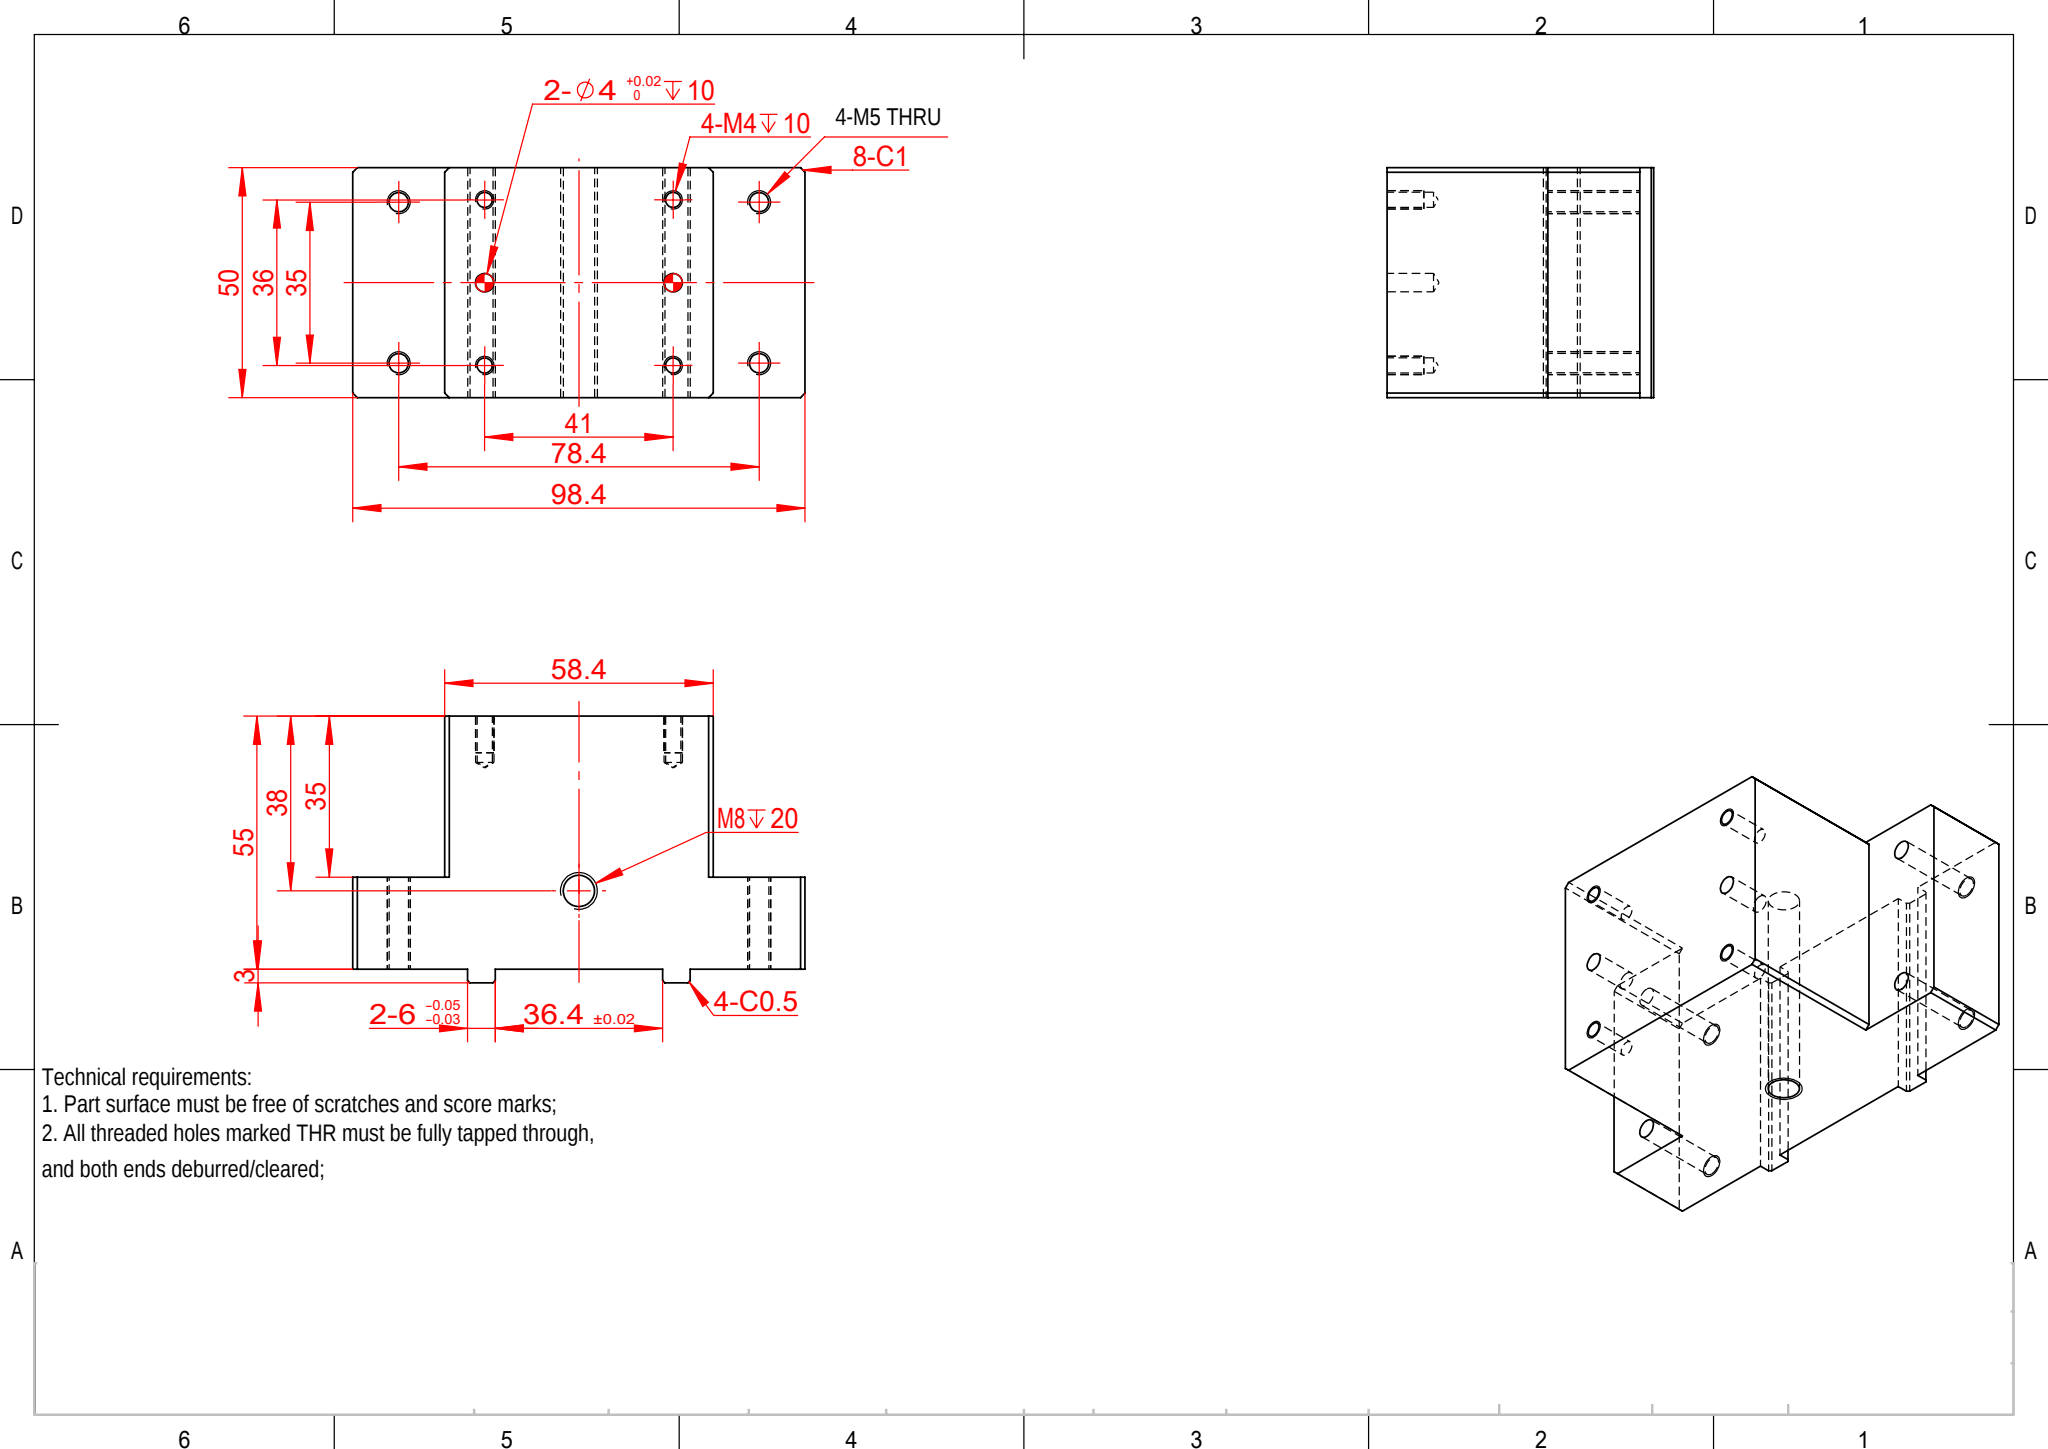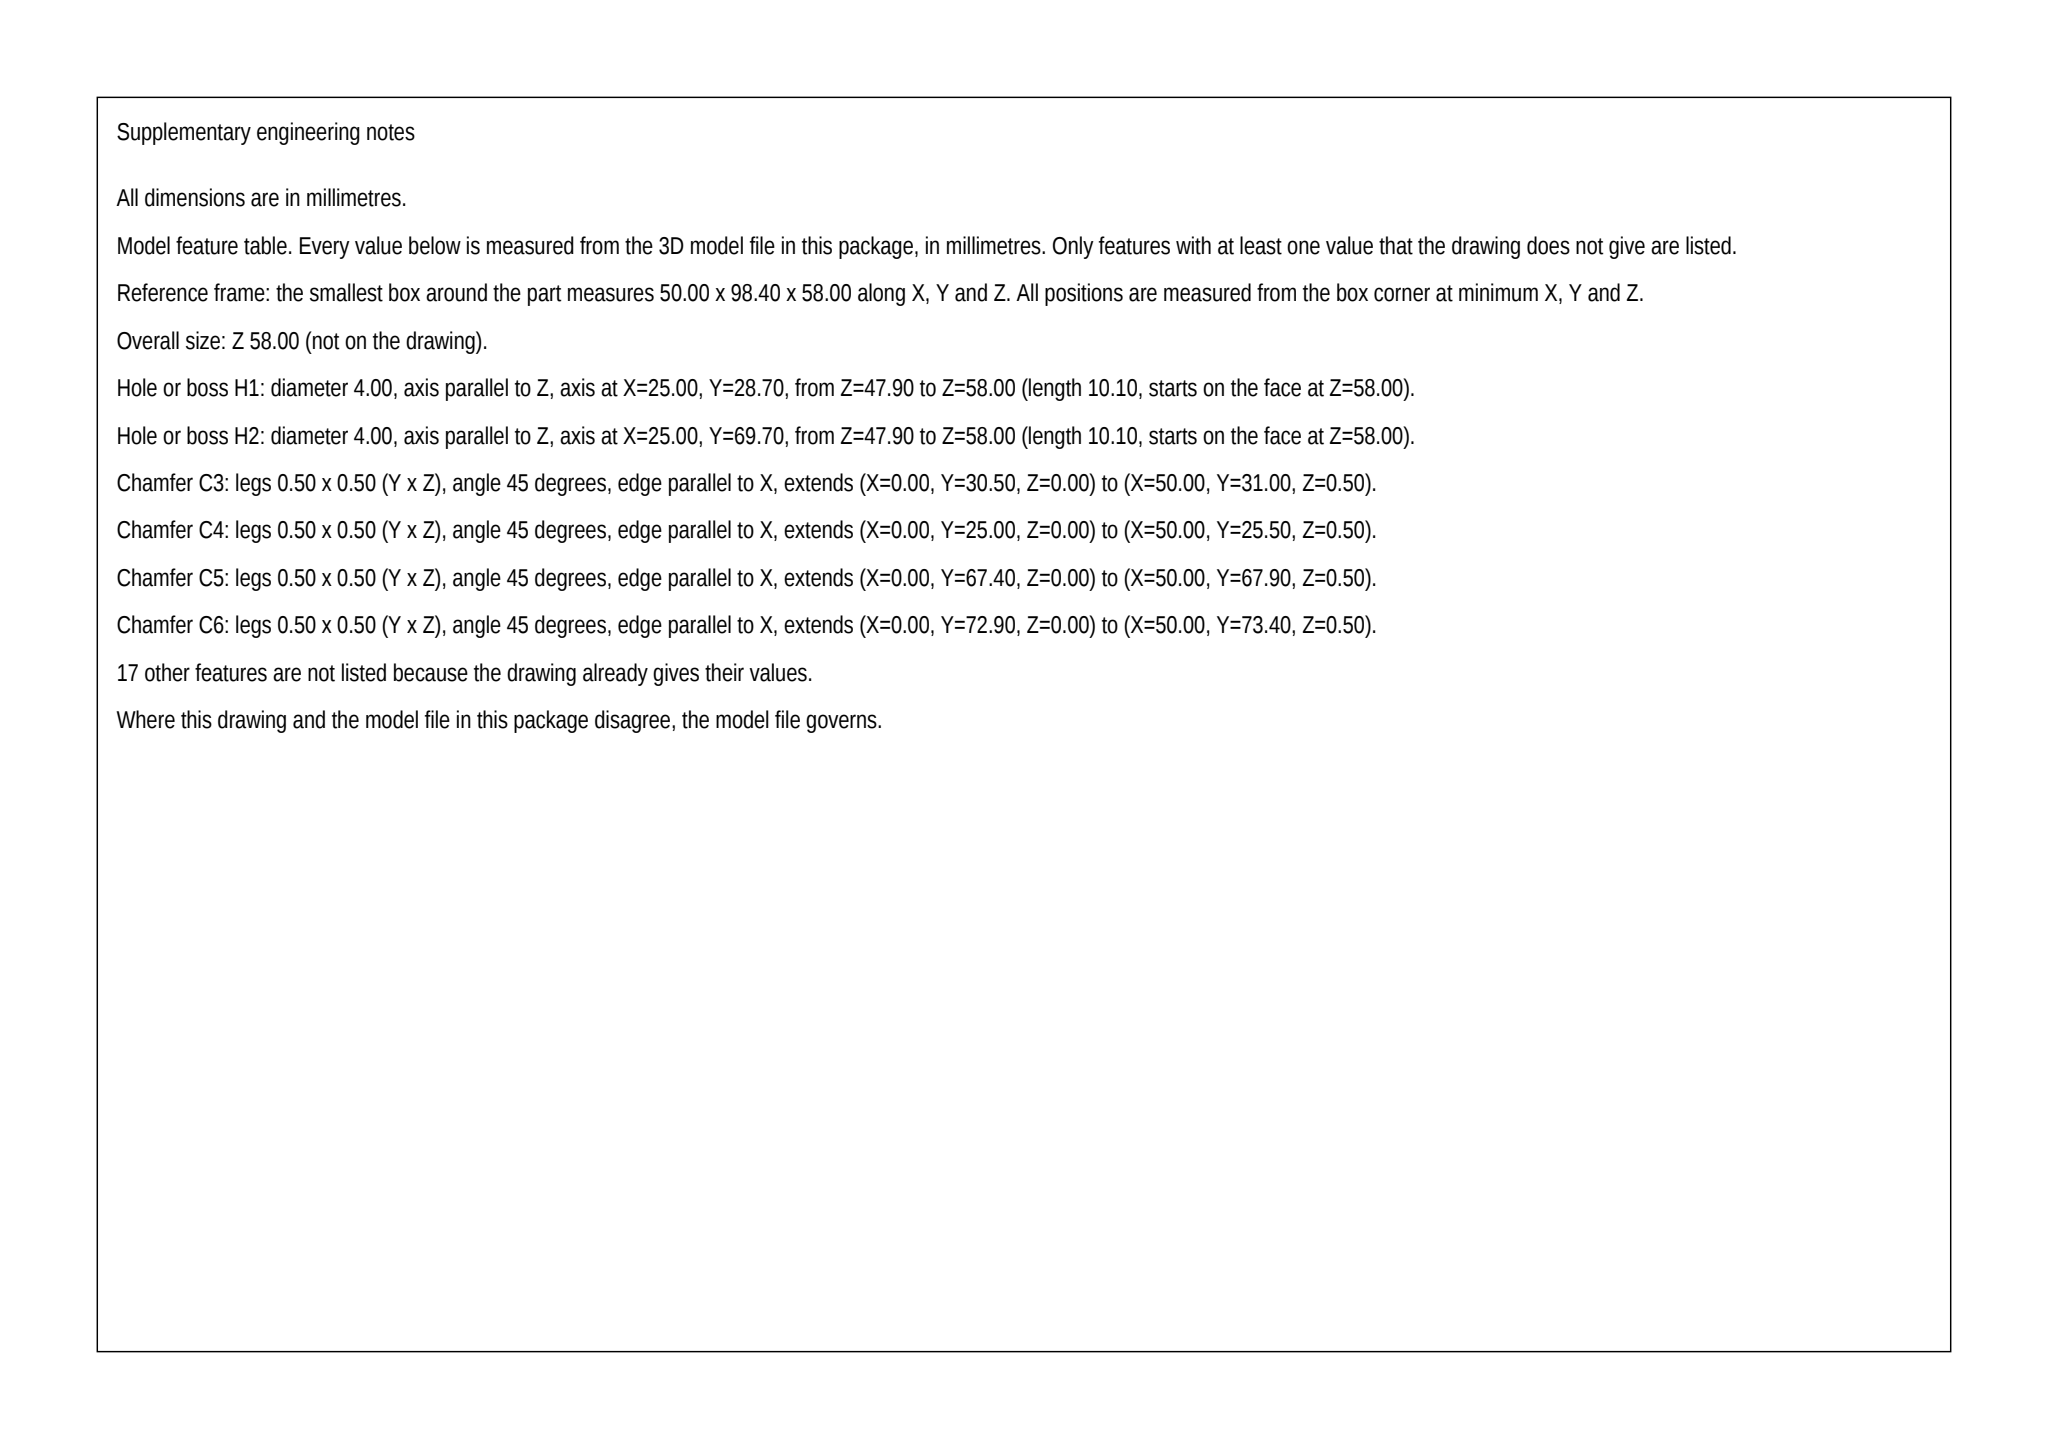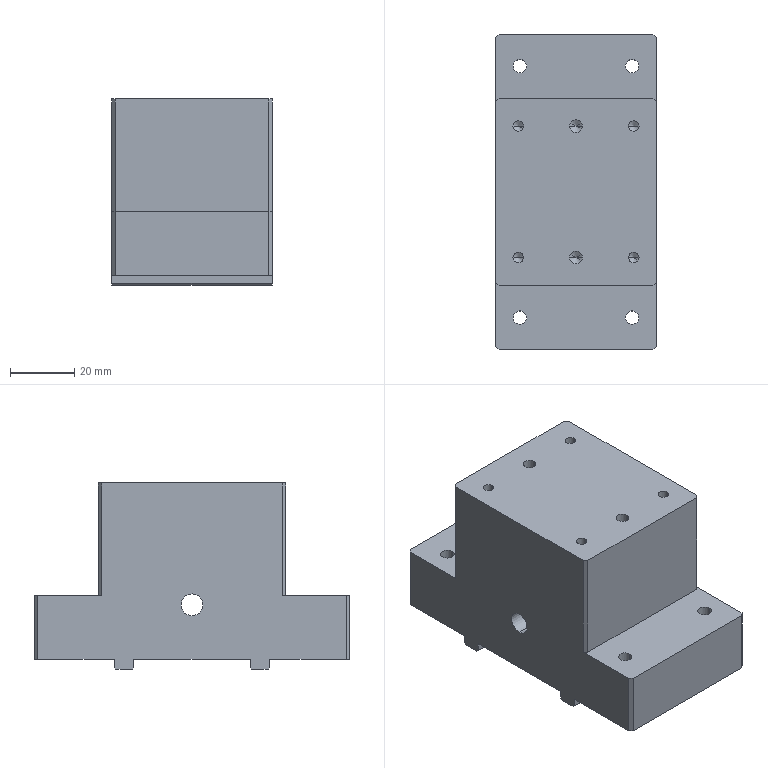Part | SolidWorks | mm | 1 solid | 64 faces | box 50 x 98.4 x 58 mm | volume 198720 mm3 | plane 30 | cylinder 22 | cone 12 | commonest cylinder face diameters 4.2 x8 3.3 x8 4 x4 6.8 x2
build123d program:
from build123d import *

# Parameters (mm, degrees)
SKETCH1_W                     = 50
SKETCH1_H                     = 98.4
BOSS_EXTRUDE1_DEPTH           = 55
SKETCH2_W                     = 35
SKETCH2_H                     = 20
CUT_EXTRUDE1_DEPTH            = 90.138
SKETCH3_W                     = 3
SKETCH3_H                     = 6
BOSS_EXTRUDE2_DEPTH           = 50
CHAMFER1_SIZE                 = 0.5
M4_TAPPED_HOLE1_D             = 3.3
M4_TAPPED_HOLE1_DEPTH         = 10.1
M4_TAPPED_HOLE1_TIP           = 0.9914
SIZE_MM_DOWEL_PIN_HOLE1_D     = 4
SIZE_MM_DOWEL_PIN_HOLE1_DEPTH = 10.1
SIZE_MM_DOWEL_PIN_HOLE1_TIP   = 1.202
M5_TAPPED_HOLE1_D             = 4.2
M8_TAPPED_HOLE1_D             = 6.8
CHAMFER2_SIZE                 = 1
CHAMFER3_SIZE                 = 1
CHAMFER1_OF_MIRROR4_SIZE      = 0.5


with BuildPart() as part:
    # Sketch1 → Boss-Extrude1 (new body)
    with BuildSketch(Plane.XY):
        Rectangle(SKETCH1_W, SKETCH1_H)
    extrude(amount=BOSS_EXTRUDE1_DEPTH)

    # Sketch2 → Cut-Extrude1 (cut, through all)
    with BuildSketch(Plane(origin=(25, 0, 0), x_dir=(0, 0, -1), z_dir=(1, 0, 0))):
        with Locations((-37.5, -39.2)):
            Rectangle(SKETCH2_W, SKETCH2_H)
    cut_extrude1 = extrude(amount=-CUT_EXTRUDE1_DEPTH, mode=Mode.SUBTRACT)

    # Mirror1: Cut-Extrude1 across plane
    add(cut_extrude1.mirror(Plane.ZX), mode=Mode.SUBTRACT)

    # Sketch3 → Boss-Extrude2 (add)
    with BuildSketch(Plane.ZY.offset(25)):
        with Locations((-1.5, -21.2)):
            Rectangle(SKETCH3_W, SKETCH3_H)
    boss_extrude2 = extrude(amount=-BOSS_EXTRUDE2_DEPTH)

    # Chamfer1
    chamfer1_edges = [part.edges().sort_by_distance(p)[0] for p in [
        (0, -24.2, -3),
        (0, -18.2, -3),
    ]]
    chamfer(chamfer1_edges, length=CHAMFER1_SIZE)

    # M4 Tapped Hole1
    with Locations(Plane.XY.offset(55)):
        with Locations((-18, -20.5), (-18, 20.5), (18, 20.5), (18, -20.5)):
            Hole(M4_TAPPED_HOLE1_D / 2, depth=M4_TAPPED_HOLE1_DEPTH)
            with Locations((0, 0, -(M4_TAPPED_HOLE1_DEPTH + M4_TAPPED_HOLE1_TIP / 2))):  # 118° drill point
                Cone(0, M4_TAPPED_HOLE1_D / 2, M4_TAPPED_HOLE1_TIP, mode=Mode.SUBTRACT)

    # Size mm Dowel Pin Hole1
    with Locations(Plane.XY.offset(55)):
        with Locations((0, -20.5), (0, 20.5)):
            Hole(SIZE_MM_DOWEL_PIN_HOLE1_D / 2, depth=SIZE_MM_DOWEL_PIN_HOLE1_DEPTH)
            with Locations((0, 0, -(SIZE_MM_DOWEL_PIN_HOLE1_DEPTH + SIZE_MM_DOWEL_PIN_HOLE1_TIP / 2))):  # 118° drill point
                Cone(0, SIZE_MM_DOWEL_PIN_HOLE1_D / 2, SIZE_MM_DOWEL_PIN_HOLE1_TIP, mode=Mode.SUBTRACT)

    # M5 Tapped Hole1 (through all)
    with Locations(Plane(origin=(0, 0, 0), x_dir=(-1, 0, 0), z_dir=(0, 0, -1))):
        with Locations((17.5, 39.2), (-17.5, 39.2)):
            m5_tapped_hole1 = Hole(M5_TAPPED_HOLE1_D / 2)

    # Mirror3: M5 Tapped Hole1 across plane
    add(m5_tapped_hole1.mirror(Plane.ZX), mode=Mode.SUBTRACT)

    # M8 Tapped Hole1 (through all)
    with Locations(Plane.ZY.offset(25)):
        with Locations((17, 0)):
            Hole(M8_TAPPED_HOLE1_D / 2)

    # Chamfer2
    chamfer2_edges = [part.edges().sort_by_distance(p)[0] for p in [
        (25, -49.2, 10),
        (-25, -49.2, 10),
        (-25, 49.2, 10),
        (25, 49.2, 10),
    ]]
    chamfer(chamfer2_edges, length=CHAMFER2_SIZE)

    # Chamfer3
    chamfer3_edges = [part.edges().sort_by_distance(p)[0] for p in [
        (-25, -29.2, 37.5),
        (25, -29.2, 37.5),
        (25, 29.2, 37.5),
        (-25, 29.2, 37.5),
    ]]
    chamfer(chamfer3_edges, length=CHAMFER3_SIZE)

    # Mirror4: Boss-Extrude2 across plane
    add(boss_extrude2.mirror(Plane.ZX))

    # Chamfer1 of Mirror4
    chamfer1_of_mirror4_edges = [part.edges().sort_by_distance(p)[0] for p in [
        (0, 24.2, -3),
        (0, 18.2, -3),
    ]]
    chamfer(chamfer1_of_mirror4_edges, length=CHAMFER1_OF_MIRROR4_SIZE)


solid = part.part